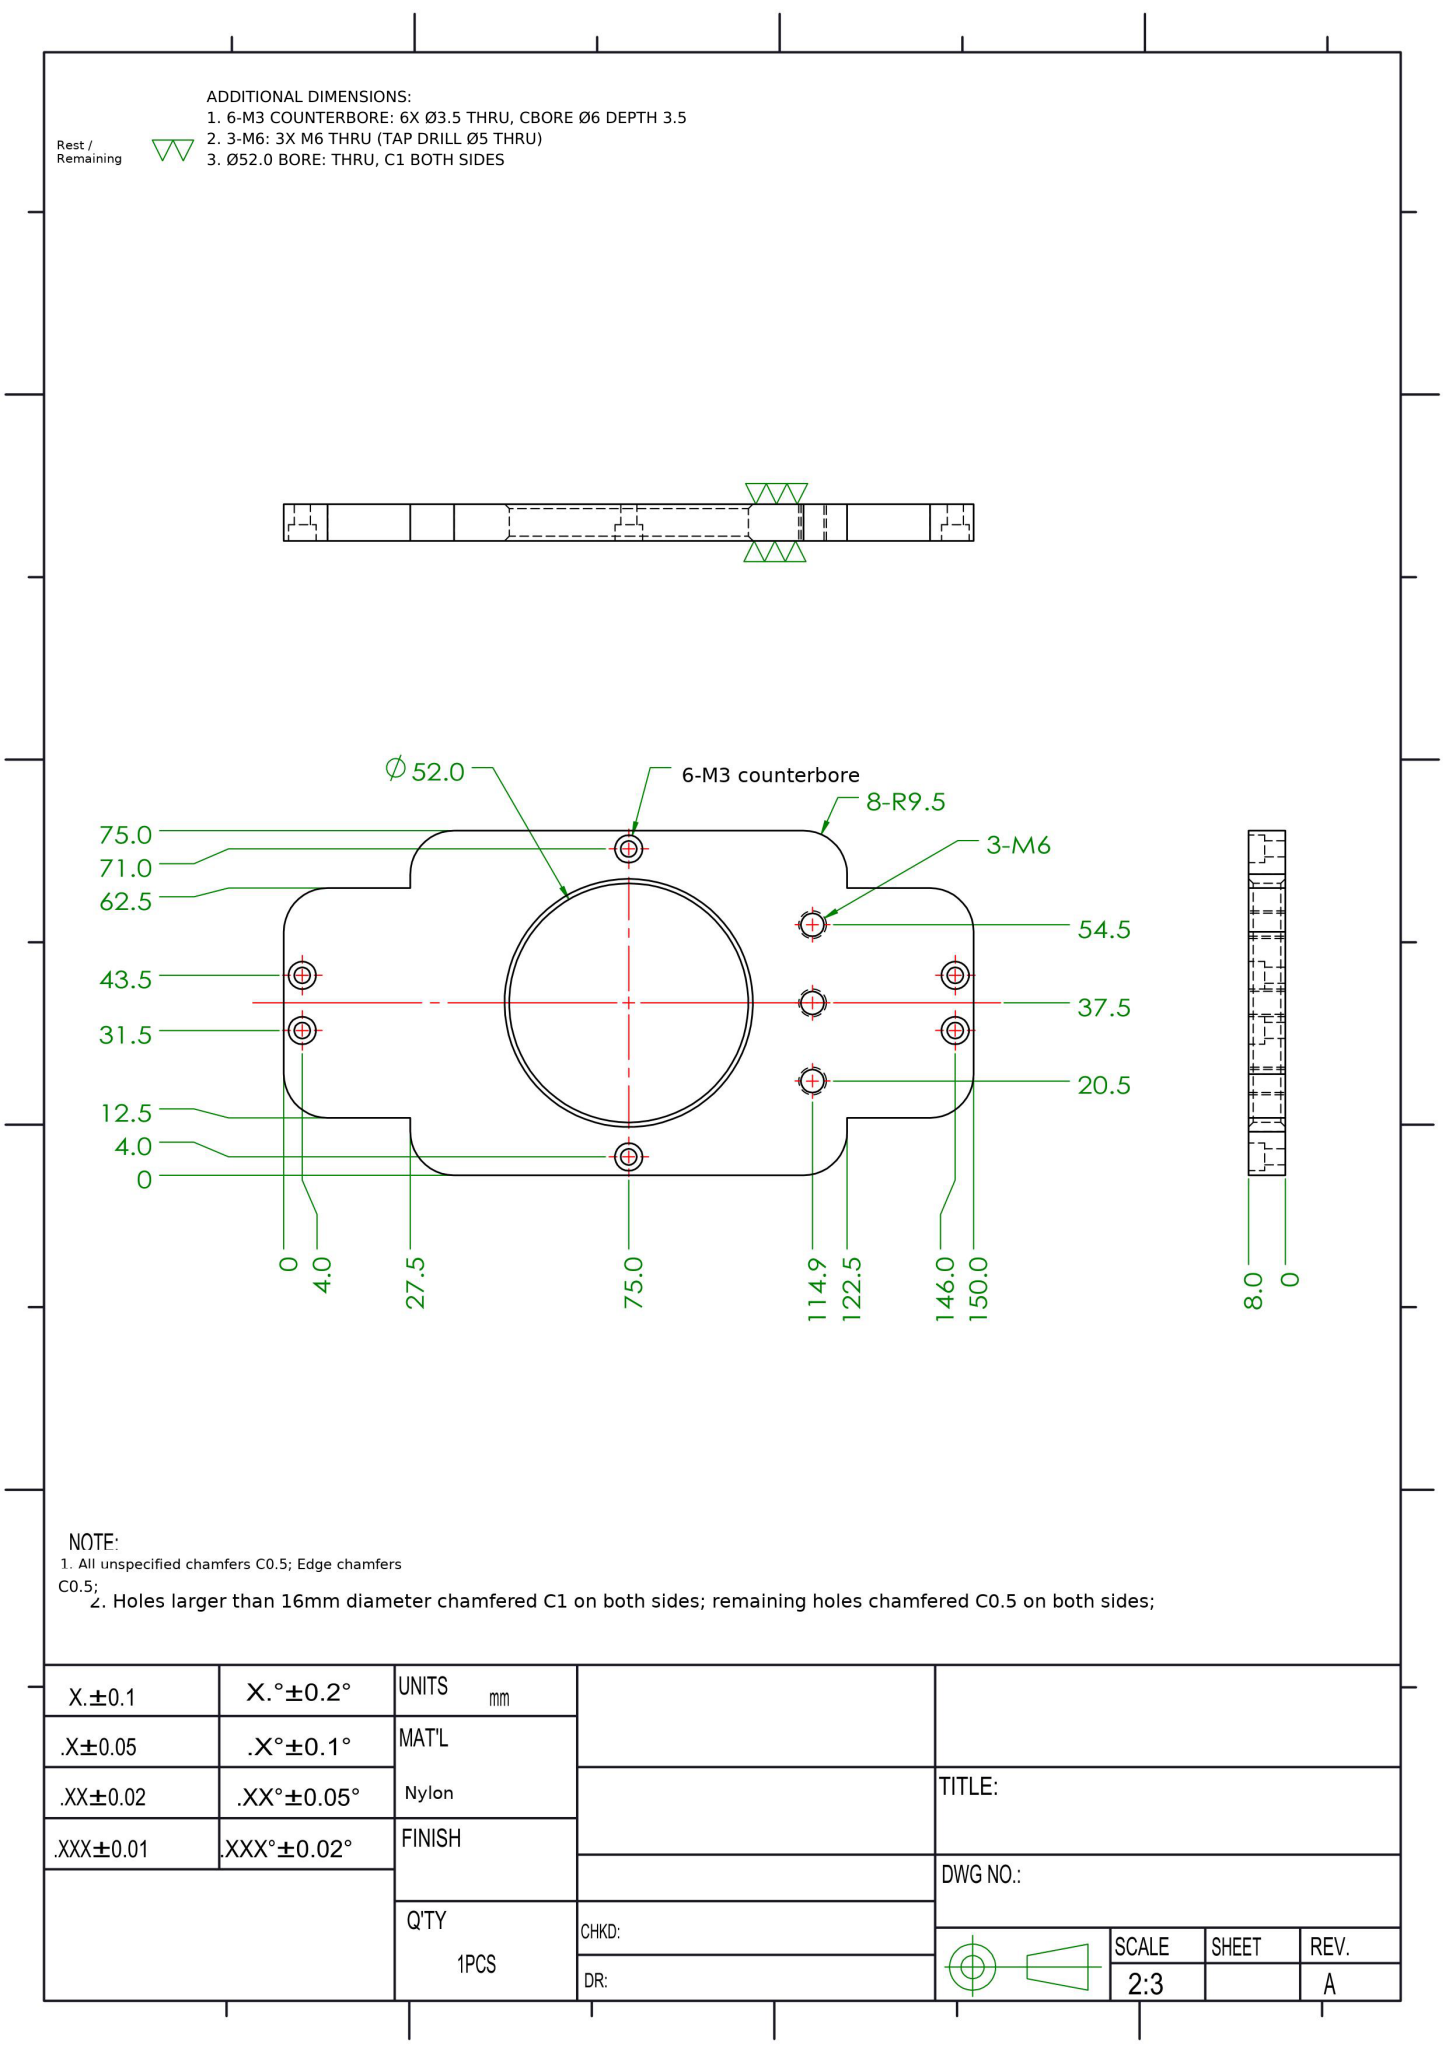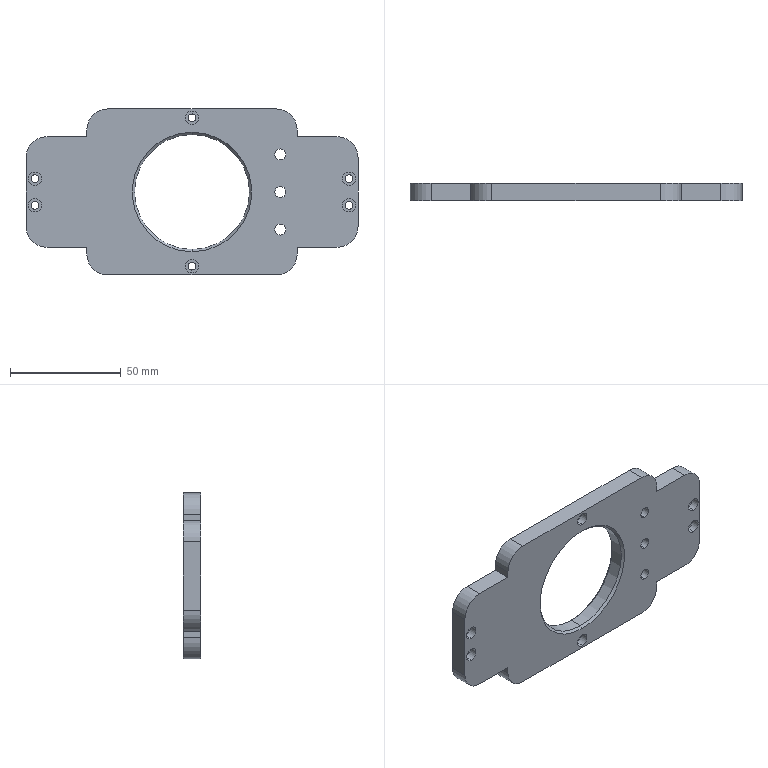Part | NX | mm | 1 solid | 64 faces | box 150 x 8 x 75 mm | volume 59280 mm3 | cylinder 40 | plane 20 | cone 4 | commonest cylinder face diameters 6 x12 3.5 x12 19 x8 5 x6 52 x2